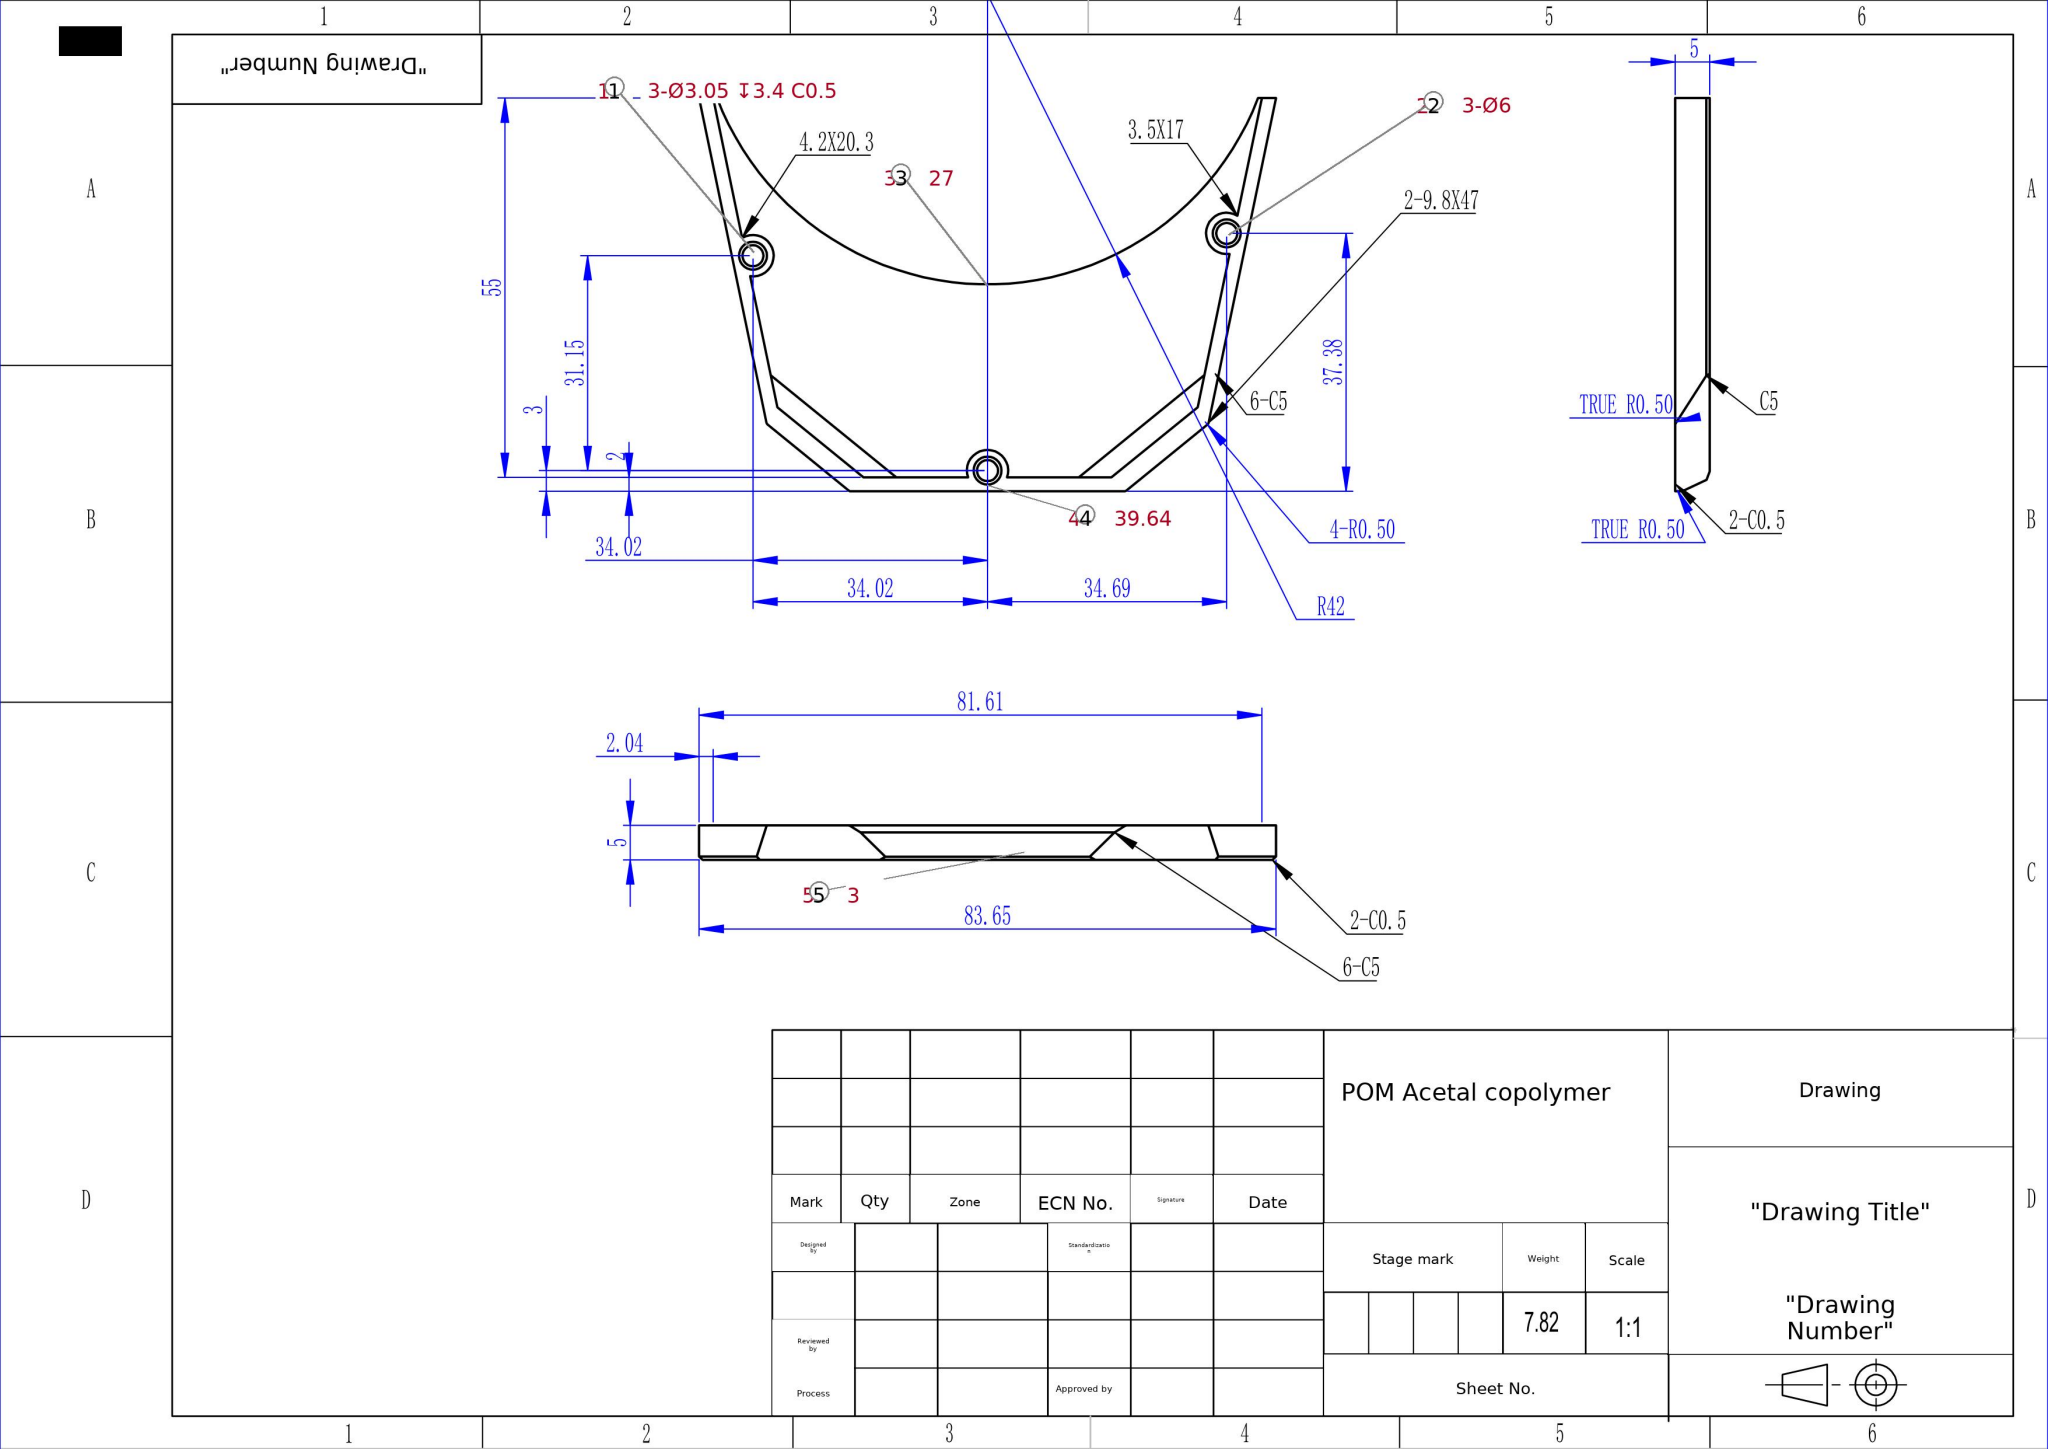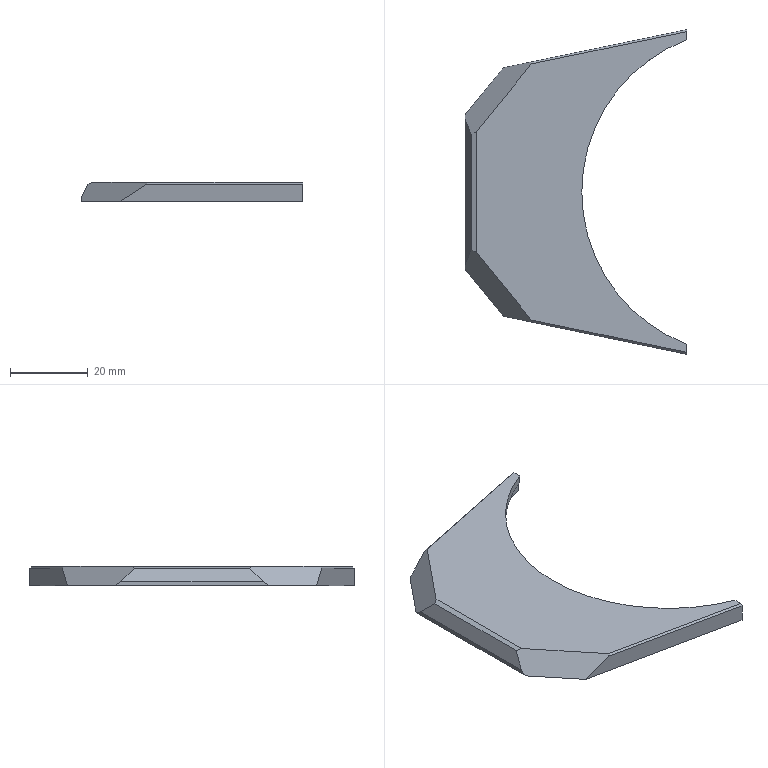Part | SolidWorks | mm | material POM Acetal copolymer | 1 solid | 49 faces | box 57 x 83.65 x 5 mm | volume 5626 mm3 | plane 25 | cylinder 18 | cone 6 | commonest cylinder face diameters 6 x7 3.05 x6 1 x4 84 x1